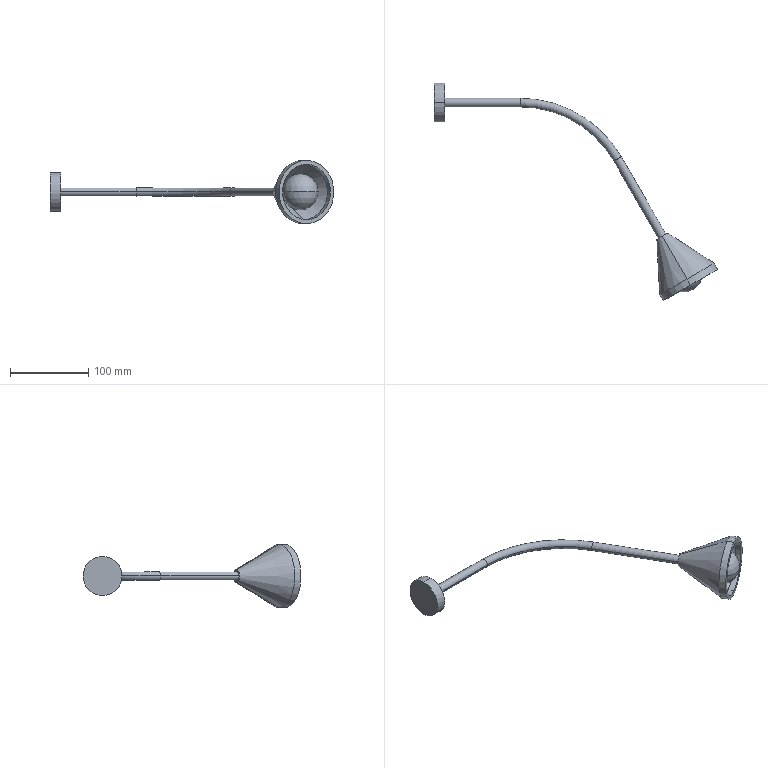Component | SolidWorks | Light-1 | 1 solid | 34 faces | box 363.07 x 279.08 x 81 mm | volume 179024 mm3 | cylinder 16 | cone 6 | plane 6 | torus 4 | sphere 2 | commonest cylinder face diameters 11 x4 1 x4 10.098 x2 71 x2 50 x2 81 x2
STEP:
#1=COLOUR_RGB('',0.7922,0.8196,0.9333);
#2=FILL_AREA_STYLE_COLOUR('',#1);
#3=FILL_AREA_STYLE('',(#2));
#4=SURFACE_STYLE_FILL_AREA(#3);
#5=SURFACE_SIDE_STYLE('',(#4));
#6=SURFACE_STYLE_USAGE(.BOTH.,#5);
#7=PRESENTATION_STYLE_ASSIGNMENT((#6));
#8=CARTESIAN_POINT('',(3.087,39.443,17.994));
#9=VERTEX_POINT('',#8);
#10=CARTESIAN_POINT('',(1.677,38.629,17.994));
#11=VERTEX_POINT('',#10);
#12=CARTESIAN_POINT('',(2.382,39.036,17.994));
#13=DIRECTION('',(0.5,-0.866,0.));
#14=DIRECTION('',(0.866,0.5,0.));
#15=AXIS2_PLACEMENT_3D('',#12,#13,#14);
#16=CIRCLE('',#15,0.8139);
#17=EDGE_CURVE('',#9,#11,#16,.T.);
#18=ORIENTED_EDGE('',*,*,#17,.T.);
#19=CARTESIAN_POINT('',(2.579,38.694,17.994));
#20=DIRECTION('',(0.,0.,-1.));
#21=DIRECTION('',(0.5611,0.8277,0.));
#22=AXIS2_PLACEMENT_3D('',#19,#20,#21);
#23=CIRCLE('',#22,0.9045);
#24=EDGE_CURVE('',#9,#11,#23,.T.);
#25=ORIENTED_EDGE('',*,*,#24,.F.);
#26=EDGE_LOOP('',(#18,#25));
#27=FACE_OUTER_BOUND('',#26,.T.);
#28=CARTESIAN_POINT('',(2.579,38.694,17.994));
#29=DIRECTION('',(0.,0.,1.));
#30=DIRECTION('',(-0.866,-0.5,0.));
#31=AXIS2_PLACEMENT_3D('',#28,#29,#30);
#32=SPHERICAL_SURFACE('',#31,0.9045);
#33=ADVANCED_FACE('',(#27),#32,.T.);
#34=ORIENTED_EDGE('',*,*,#24,.T.);
#35=CARTESIAN_POINT('',(2.382,39.036,17.994));
#36=DIRECTION('',(-0.5,0.866,0.));
#37=DIRECTION('',(0.866,0.5,0.));
#38=AXIS2_PLACEMENT_3D('',#35,#36,#37);
#39=CIRCLE('',#38,0.8139);
#40=EDGE_CURVE('',#9,#11,#39,.T.);
#41=ORIENTED_EDGE('',*,*,#40,.F.);
#42=EDGE_LOOP('',(#34,#41));
#43=FACE_OUTER_BOUND('',#42,.T.);
#44=CARTESIAN_POINT('',(2.579,38.694,17.994));
#45=DIRECTION('',(0.,0.,1.));
#46=DIRECTION('',(-0.866,-0.5,0.));
#47=AXIS2_PLACEMENT_3D('',#44,#45,#46);
#48=SPHERICAL_SURFACE('',#47,0.9045);
#49=ADVANCED_FACE('',(#43),#48,.T.);
#50=ORIENTED_EDGE('',*,*,#40,.T.);
#51=CARTESIAN_POINT('',(1.576,40.035,17.994));
#52=VERTEX_POINT('',#51);
#53=CARTESIAN_POINT('',(1.576,40.035,17.994));
#54=DIRECTION('',(0.07208,-0.9974,0.));
#55=VECTOR('',#54,39.37);
#56=LINE('',#53,#55);
#57=EDGE_CURVE('',#52,#11,#56,.T.);
#58=ORIENTED_EDGE('',*,*,#57,.F.);
#59=CARTESIAN_POINT('',(1.92,40.234,17.994));
#60=VERTEX_POINT('',#59);
#61=CARTESIAN_POINT('',(1.748,40.135,17.994));
#62=DIRECTION('',(-0.5,0.866,0.));
#63=DIRECTION('',(0.866,0.5,0.));
#64=AXIS2_PLACEMENT_3D('',#61,#62,#63);
#65=CIRCLE('',#64,0.1988);
#66=EDGE_CURVE('',#60,#52,#65,.T.);
#67=ORIENTED_EDGE('',*,*,#66,.F.);
#68=CARTESIAN_POINT('',(1.92,40.234,17.994));
#69=DIRECTION('',(0.8277,-0.5611,0.));
#70=VECTOR('',#69,39.37);
#71=LINE('',#68,#70);
#72=EDGE_CURVE('',#60,#9,#71,.T.);
#73=ORIENTED_EDGE('',*,*,#72,.T.);
#74=EDGE_LOOP('',(#50,#58,#67,#73));
#75=FACE_OUTER_BOUND('',#74,.T.);
#76=CARTESIAN_POINT('',(1.735,40.157,17.994));
#77=DIRECTION('',(0.5,-0.866,0.));
#78=DIRECTION('',(0.866,0.5,0.));
#79=AXIS2_PLACEMENT_3D('',#76,#77,#78);
#80=CONICAL_SURFACE('',#79,0.1865,0.4515);
#81=ADVANCED_FACE('',(#75),#80,.T.);
#82=CARTESIAN_POINT('',(1.748,40.135,17.994));
#83=DIRECTION('',(0.5,-0.866,0.));
#84=DIRECTION('',(0.866,0.5,0.));
#85=AXIS2_PLACEMENT_3D('',#82,#83,#84);
#86=CIRCLE('',#85,0.1988);
#87=EDGE_CURVE('',#60,#52,#86,.T.);
#88=ORIENTED_EDGE('',*,*,#87,.T.);
#89=ORIENTED_EDGE('',*,*,#57,.T.);
#90=ORIENTED_EDGE('',*,*,#17,.F.);
#91=ORIENTED_EDGE('',*,*,#72,.F.);
#92=EDGE_LOOP('',(#88,#89,#90,#91));
#93=FACE_OUTER_BOUND('',#92,.T.);
#94=CARTESIAN_POINT('',(1.735,40.157,17.994));
#95=DIRECTION('',(0.5,-0.866,0.));
#96=DIRECTION('',(0.866,0.5,0.));
#97=AXIS2_PLACEMENT_3D('',#94,#95,#96);
#98=CONICAL_SURFACE('',#97,0.1865,0.4515);
#99=ADVANCED_FACE('',(#93),#98,.T.);
#100=CARTESIAN_POINT('',(1.409,40.324,17.994));
#101=VERTEX_POINT('',#100);
#102=CARTESIAN_POINT('',(1.409,40.324,17.994));
#103=DIRECTION('',(0.5,-0.866,0.));
#104=VECTOR('',#103,39.37);
#105=LINE('',#102,#104);
#106=EDGE_CURVE('',#101,#52,#105,.T.);
#107=ORIENTED_EDGE('',*,*,#106,.T.);
#108=ORIENTED_EDGE('',*,*,#87,.F.);
#109=CARTESIAN_POINT('',(1.754,40.522,17.994));
#110=VERTEX_POINT('',#109);
#111=CARTESIAN_POINT('',(1.754,40.522,17.994));
#112=DIRECTION('',(0.5,-0.866,0.));
#113=VECTOR('',#112,39.37);
#114=LINE('',#111,#113);
#115=EDGE_CURVE('',#110,#60,#114,.T.);
#116=ORIENTED_EDGE('',*,*,#115,.F.);
#117=CARTESIAN_POINT('',(1.581,40.423,18.193));
#118=VERTEX_POINT('',#117);
#119=CARTESIAN_POINT('',(1.581,40.423,17.994));
#120=DIRECTION('',(-0.5,0.866,0.));
#121=DIRECTION('',(-0.00000001,-0.00000001,1.));
#122=AXIS2_PLACEMENT_3D('',#119,#120,#121);
#123=CIRCLE('',#122,0.1988);
#124=EDGE_CURVE('',#118,#110,#123,.T.);
#125=ORIENTED_EDGE('',*,*,#124,.F.);
#126=CARTESIAN_POINT('',(1.581,40.423,17.994));
#127=DIRECTION('',(-0.5,0.866,0.));
#128=DIRECTION('',(-0.866,-0.5,0.));
#129=AXIS2_PLACEMENT_3D('',#126,#127,#128);
#130=CIRCLE('',#129,0.1988);
#131=EDGE_CURVE('',#101,#118,#130,.T.);
#132=ORIENTED_EDGE('',*,*,#131,.F.);
#133=EDGE_LOOP('',(#107,#108,#116,#125,#132));
#134=FACE_OUTER_BOUND('',#133,.T.);
#135=CARTESIAN_POINT('',(3.225,37.576,17.994));
#136=DIRECTION('',(-0.5,0.866,0.));
#137=DIRECTION('',(-0.866,-0.5,0.));
#138=AXIS2_PLACEMENT_3D('',#135,#136,#137);
#139=CYLINDRICAL_SURFACE('',#138,0.1988);
#140=ADVANCED_FACE('',(#134),#139,.T.);
#141=ORIENTED_EDGE('',*,*,#131,.T.);
#142=CARTESIAN_POINT('',(2.747,38.404,19.392));
#143=VERTEX_POINT('',#142);
#144=CARTESIAN_POINT('',(1.581,40.423,18.193));
#145=DIRECTION('',(0.4446,-0.7701,0.4573));
#146=VECTOR('',#145,39.37);
#147=LINE('',#144,#146);
#148=EDGE_CURVE('',#118,#143,#147,.T.);
#149=ORIENTED_EDGE('',*,*,#148,.T.);
#150=CARTESIAN_POINT('',(2.747,38.404,16.597));
#151=VERTEX_POINT('',#150);
#152=CARTESIAN_POINT('',(2.747,38.404,17.994));
#153=DIRECTION('',(-0.5,0.866,0.));
#154=DIRECTION('',(0.,0.,-1.));
#155=AXIS2_PLACEMENT_3D('',#152,#153,#154);
#156=CIRCLE('',#155,1.398);
#157=EDGE_CURVE('',#151,#143,#156,.T.);
#158=ORIENTED_EDGE('',*,*,#157,.F.);
#159=CARTESIAN_POINT('',(1.581,40.423,17.796));
#160=VERTEX_POINT('',#159);
#161=CARTESIAN_POINT('',(1.581,40.423,17.796));
#162=DIRECTION('',(0.4446,-0.7701,-0.4573));
#163=VECTOR('',#162,39.37);
#164=LINE('',#161,#163);
#165=EDGE_CURVE('',#160,#151,#164,.T.);
#166=ORIENTED_EDGE('',*,*,#165,.F.);
#167=CARTESIAN_POINT('',(1.581,40.423,17.994));
#168=DIRECTION('',(-0.5,0.866,0.));
#169=DIRECTION('',(0.00000001,0.00000001,-1.));
#170=AXIS2_PLACEMENT_3D('',#167,#168,#169);
#171=CIRCLE('',#170,0.1988);
#172=EDGE_CURVE('',#160,#101,#171,.T.);
#173=ORIENTED_EDGE('',*,*,#172,.T.);
#174=EDGE_LOOP('',(#141,#149,#158,#166,#173));
#175=FACE_OUTER_BOUND('',#174,.T.);
#176=CARTESIAN_POINT('',(1.558,40.463,17.994));
#177=DIRECTION('',(0.5,-0.866,0.));
#178=DIRECTION('',(0.,0.,1.));
#179=AXIS2_PLACEMENT_3D('',#176,#177,#178);
#180=CONICAL_SURFACE('',#179,0.1748,0.475);
#181=ADVANCED_FACE('',(#175),#180,.F.);
#182=ORIENTED_EDGE('',*,*,#115,.T.);
#183=ORIENTED_EDGE('',*,*,#66,.T.);
#184=ORIENTED_EDGE('',*,*,#106,.F.);
#185=ORIENTED_EDGE('',*,*,#172,.F.);
#186=CARTESIAN_POINT('',(1.581,40.423,17.994));
#187=DIRECTION('',(-0.5,0.866,0.));
#188=DIRECTION('',(0.866,0.5,0.));
#189=AXIS2_PLACEMENT_3D('',#186,#187,#188);
#190=CIRCLE('',#189,0.1988);
#191=EDGE_CURVE('',#110,#160,#190,.T.);
#192=ORIENTED_EDGE('',*,*,#191,.F.);
#193=EDGE_LOOP('',(#182,#183,#184,#185,#192));
#194=FACE_OUTER_BOUND('',#193,.T.);
#195=CARTESIAN_POINT('',(3.225,37.576,17.994));
#196=DIRECTION('',(-0.5,0.866,0.));
#197=DIRECTION('',(-0.866,-0.5,0.));
#198=AXIS2_PLACEMENT_3D('',#195,#196,#197);
#199=CYLINDRICAL_SURFACE('',#198,0.1988);
#200=ADVANCED_FACE('',(#194),#199,.T.);
#201=ORIENTED_EDGE('',*,*,#165,.T.);
#202=CARTESIAN_POINT('',(2.747,38.404,17.994));
#203=DIRECTION('',(-0.5,0.866,0.));
#204=DIRECTION('',(0.00000001,0.,1.));
#205=AXIS2_PLACEMENT_3D('',#202,#203,#204);
#206=CIRCLE('',#205,1.398);
#207=EDGE_CURVE('',#143,#151,#206,.T.);
#208=ORIENTED_EDGE('',*,*,#207,.F.);
#209=ORIENTED_EDGE('',*,*,#148,.F.);
#210=ORIENTED_EDGE('',*,*,#124,.T.);
#211=ORIENTED_EDGE('',*,*,#191,.T.);
#212=EDGE_LOOP('',(#201,#208,#209,#210,#211));
#213=FACE_OUTER_BOUND('',#212,.T.);
#214=CARTESIAN_POINT('',(1.558,40.463,17.994));
#215=DIRECTION('',(0.5,-0.866,0.));
#216=DIRECTION('',(0.,0.,1.));
#217=AXIS2_PLACEMENT_3D('',#214,#215,#216);
#218=CONICAL_SURFACE('',#217,0.1748,0.475);
#219=ADVANCED_FACE('',(#213),#218,.F.);
#220=CARTESIAN_POINT('',(2.9,38.139,19.392));
#221=VERTEX_POINT('',#220);
#222=CARTESIAN_POINT('',(2.9,38.139,19.392));
#223=DIRECTION('',(-0.5,0.866,0.));
#224=VECTOR('',#223,39.37);
#225=LINE('',#222,#224);
#226=EDGE_CURVE('',#221,#143,#225,.T.);
#227=ORIENTED_EDGE('',*,*,#226,.T.);
#228=ORIENTED_EDGE('',*,*,#207,.T.);
#229=CARTESIAN_POINT('',(2.9,38.139,16.597));
#230=VERTEX_POINT('',#229);
#231=CARTESIAN_POINT('',(2.9,38.139,16.597));
#232=DIRECTION('',(-0.5,0.866,0.));
#233=VECTOR('',#232,39.37);
#234=LINE('',#231,#233);
#235=EDGE_CURVE('',#230,#151,#234,.T.);
#236=ORIENTED_EDGE('',*,*,#235,.F.);
#237=CARTESIAN_POINT('',(2.9,38.139,17.994));
#238=DIRECTION('',(0.5,-0.866,0.));
#239=DIRECTION('',(0.,0.,-1.));
#240=AXIS2_PLACEMENT_3D('',#237,#238,#239);
#241=CIRCLE('',#240,1.398);
#242=EDGE_CURVE('',#230,#221,#241,.T.);
#243=ORIENTED_EDGE('',*,*,#242,.T.);
#244=EDGE_LOOP('',(#227,#228,#236,#243));
#245=FACE_OUTER_BOUND('',#244,.T.);
#246=CARTESIAN_POINT('',(2.9,38.139,17.994));
#247=DIRECTION('',(0.5,-0.866,0.));
#248=DIRECTION('',(0.,0.,-1.));
#249=AXIS2_PLACEMENT_3D('',#246,#247,#248);
#250=CYLINDRICAL_SURFACE('',#249,1.398);
#251=ADVANCED_FACE('',(#245),#250,.F.);
#252=CARTESIAN_POINT('',(-5.688,47.561,17.994));
#253=VERTEX_POINT('',#252);
#254=CARTESIAN_POINT('',(-0.5905,44.618,17.994));
#255=VERTEX_POINT('',#254);
#256=CARTESIAN_POINT('',(-5.688,41.675,17.994));
#257=DIRECTION('',(0.,0.,-1.));
#258=DIRECTION('',(0.,1.,0.));
#259=AXIS2_PLACEMENT_3D('',#256,#257,#258);
#260=CIRCLE('',#259,5.886);
#261=EDGE_CURVE('',#253,#255,#260,.T.);
#262=ORIENTED_EDGE('',*,*,#261,.T.);
#263=CARTESIAN_POINT('',(-0.9656,44.401,17.994));
#264=VERTEX_POINT('',#263);
#265=CARTESIAN_POINT('',(-0.7781,44.51,17.994));
#266=DIRECTION('',(0.5,-0.866,0.));
#267=DIRECTION('',(-0.866,-0.5,0.));
#268=AXIS2_PLACEMENT_3D('',#265,#266,#267);
#269=CIRCLE('',#268,0.2165);
#270=EDGE_CURVE('',#264,#255,#269,.T.);
#271=ORIENTED_EDGE('',*,*,#270,.F.);
#272=CARTESIAN_POINT('',(-5.688,47.128,17.994));
#273=VERTEX_POINT('',#272);
#274=CARTESIAN_POINT('',(-5.688,41.675,17.994));
#275=DIRECTION('',(0.,0.,-1.));
#276=DIRECTION('',(0.,1.,0.));
#277=AXIS2_PLACEMENT_3D('',#274,#275,#276);
#278=CIRCLE('',#277,5.453);
#279=EDGE_CURVE('',#273,#264,#278,.T.);
#280=ORIENTED_EDGE('',*,*,#279,.F.);
#281=CARTESIAN_POINT('',(-5.688,47.344,17.994));
#282=DIRECTION('',(1.,0.,0.));
#283=DIRECTION('',(0.,-1.,0.));
#284=AXIS2_PLACEMENT_3D('',#281,#282,#283);
#285=CIRCLE('',#284,0.2165);
#286=EDGE_CURVE('',#273,#253,#285,.T.);
#287=ORIENTED_EDGE('',*,*,#286,.T.);
#288=EDGE_LOOP('',(#262,#271,#280,#287));
#289=FACE_OUTER_BOUND('',#288,.T.);
#290=CARTESIAN_POINT('',(-5.688,41.675,17.994));
#291=DIRECTION('',(0.,0.,-1.));
#292=DIRECTION('',(0.,-1.,0.));
#293=AXIS2_PLACEMENT_3D('',#290,#291,#292);
#294=TOROIDAL_SURFACE('',#293,5.669,0.2165);
#295=ADVANCED_FACE('',(#289),#294,.T.);
#296=CARTESIAN_POINT('',(-9.501,47.561,17.994));
#297=VERTEX_POINT('',#296);
#298=CARTESIAN_POINT('',(-9.501,47.561,17.994));
#299=DIRECTION('',(1.,0.,0.));
#300=VECTOR('',#299,39.37);
#301=LINE('',#298,#300);
#302=EDGE_CURVE('',#297,#253,#301,.T.);
#303=ORIENTED_EDGE('',*,*,#302,.T.);
#304=ORIENTED_EDGE('',*,*,#286,.F.);
#305=CARTESIAN_POINT('',(-9.501,47.128,17.994));
#306=VERTEX_POINT('',#305);
#307=CARTESIAN_POINT('',(-9.501,47.128,17.994));
#308=DIRECTION('',(1.,0.,0.));
#309=VECTOR('',#308,39.37);
#310=LINE('',#307,#309);
#311=EDGE_CURVE('',#306,#273,#310,.T.);
#312=ORIENTED_EDGE('',*,*,#311,.F.);
#313=CARTESIAN_POINT('',(-9.501,47.344,17.994));
#314=DIRECTION('',(1.,0.,0.));
#315=DIRECTION('',(0.,-1.,0.));
#316=AXIS2_PLACEMENT_3D('',#313,#314,#315);
#317=CIRCLE('',#316,0.2165);
#318=EDGE_CURVE('',#306,#297,#317,.T.);
#319=ORIENTED_EDGE('',*,*,#318,.T.);
#320=EDGE_LOOP('',(#303,#304,#312,#319));
#321=FACE_OUTER_BOUND('',#320,.T.);
#322=CARTESIAN_POINT('',(-9.501,47.344,17.994));
#323=DIRECTION('',(1.,0.,0.));
#324=DIRECTION('',(0.,-1.,0.));
#325=AXIS2_PLACEMENT_3D('',#322,#323,#324);
#326=CYLINDRICAL_SURFACE('',#325,0.2165);
#327=ADVANCED_FACE('',(#321),#326,.T.);
#328=CARTESIAN_POINT('',(-10.013,47.344,17.01));
#329=VERTEX_POINT('',#328);
#330=CARTESIAN_POINT('',(-10.013,47.344,18.979));
#331=VERTEX_POINT('',#330);
#332=CARTESIAN_POINT('',(-10.013,47.344,17.994));
#333=DIRECTION('',(-1.,0.,0.));
#334=DIRECTION('',(0.,0.,-1.));
#335=AXIS2_PLACEMENT_3D('',#332,#333,#334);
#336=CIRCLE('',#335,0.9843);
#337=EDGE_CURVE('',#329,#331,#336,.T.);
#338=ORIENTED_EDGE('',*,*,#337,.T.);
#339=CARTESIAN_POINT('',(-10.013,47.344,17.994));
#340=DIRECTION('',(-1.,0.,0.));
#341=DIRECTION('',(0.,0.,1.));
#342=AXIS2_PLACEMENT_3D('',#339,#340,#341);
#343=CIRCLE('',#342,0.9843);
#344=EDGE_CURVE('',#331,#329,#343,.T.);
#345=ORIENTED_EDGE('',*,*,#344,.T.);
#346=EDGE_LOOP('',(#338,#345));
#347=FACE_OUTER_BOUND('',#346,.T.);
#348=CARTESIAN_POINT('',(-10.013,47.344,17.994));
#349=DIRECTION('',(-1.,0.,0.));
#350=DIRECTION('',(0.,0.,1.));
#351=AXIS2_PLACEMENT_3D('',#348,#349,#350);
#352=PLANE('',#351);
#353=ADVANCED_FACE('',(#347),#352,.T.);
#354=CARTESIAN_POINT('',(-9.501,47.344,18.979));
#355=VERTEX_POINT('',#354);
#356=CARTESIAN_POINT('',(-9.501,47.344,18.979));
#357=DIRECTION('',(-1.,0.,0.));
#358=VECTOR('',#357,39.37);
#359=LINE('',#356,#358);
#360=EDGE_CURVE('',#355,#331,#359,.T.);
#361=ORIENTED_EDGE('',*,*,#360,.T.);
#362=ORIENTED_EDGE('',*,*,#337,.F.);
#363=CARTESIAN_POINT('',(-9.501,47.344,17.01));
#364=VERTEX_POINT('',#363);
#365=CARTESIAN_POINT('',(-9.501,47.344,17.01));
#366=DIRECTION('',(-1.,0.,0.));
#367=VECTOR('',#366,39.37);
#368=LINE('',#365,#367);
#369=EDGE_CURVE('',#364,#329,#368,.T.);
#370=ORIENTED_EDGE('',*,*,#369,.F.);
#371=CARTESIAN_POINT('',(-9.501,47.344,17.994));
#372=DIRECTION('',(-1.,0.,0.));
#373=DIRECTION('',(0.,0.,-1.));
#374=AXIS2_PLACEMENT_3D('',#371,#372,#373);
#375=CIRCLE('',#374,0.9843);
#376=EDGE_CURVE('',#364,#355,#375,.T.);
#377=ORIENTED_EDGE('',*,*,#376,.T.);
#378=EDGE_LOOP('',(#361,#362,#370,#377));
#379=FACE_OUTER_BOUND('',#378,.T.);
#380=CARTESIAN_POINT('',(-9.501,47.344,17.994));
#381=DIRECTION('',(-1.,0.,0.));
#382=DIRECTION('',(0.,0.,1.));
#383=AXIS2_PLACEMENT_3D('',#380,#381,#382);
#384=CYLINDRICAL_SURFACE('',#383,0.9843);
#385=ADVANCED_FACE('',(#379),#384,.T.);
#386=ORIENTED_EDGE('',*,*,#369,.T.);
#387=ORIENTED_EDGE('',*,*,#344,.F.);
#388=ORIENTED_EDGE('',*,*,#360,.F.);
#389=CARTESIAN_POINT('',(-9.501,47.344,17.994));
#390=DIRECTION('',(-1.,0.,0.));
#391=DIRECTION('',(0.,0.,1.));
#392=AXIS2_PLACEMENT_3D('',#389,#390,#391);
#393=CIRCLE('',#392,0.9843);
#394=EDGE_CURVE('',#355,#364,#393,.T.);
#395=ORIENTED_EDGE('',*,*,#394,.T.);
#396=EDGE_LOOP('',(#386,#387,#388,#395));
#397=FACE_OUTER_BOUND('',#396,.T.);
#398=CARTESIAN_POINT('',(-9.501,47.344,17.994));
#399=DIRECTION('',(-1.,0.,0.));
#400=DIRECTION('',(0.,0.,1.));
#401=AXIS2_PLACEMENT_3D('',#398,#399,#400);
#402=CYLINDRICAL_SURFACE('',#401,0.9843);
#403=ADVANCED_FACE('',(#397),#402,.T.);
#404=CARTESIAN_POINT('',(-9.501,47.344,17.994));
#405=DIRECTION('',(1.,0.,0.));
#406=DIRECTION('',(0.,1.,0.));
#407=AXIS2_PLACEMENT_3D('',#404,#405,#406);
#408=CIRCLE('',#407,0.2165);
#409=EDGE_CURVE('',#297,#306,#408,.T.);
#410=ORIENTED_EDGE('',*,*,#409,.F.);
#411=ORIENTED_EDGE('',*,*,#318,.F.);
#412=EDGE_LOOP('',(#410,#411));
#413=FACE_BOUND('',#412,.T.);
#414=ORIENTED_EDGE('',*,*,#376,.F.);
#415=ORIENTED_EDGE('',*,*,#394,.F.);
#416=EDGE_LOOP('',(#414,#415));
#417=FACE_OUTER_BOUND('',#416,.T.);
#418=CARTESIAN_POINT('',(-9.501,47.344,17.994));
#419=DIRECTION('',(-1.,0.,0.));
#420=DIRECTION('',(0.,0.,1.));
#421=AXIS2_PLACEMENT_3D('',#418,#419,#420);
#422=PLANE('',#421);
#423=ADVANCED_FACE('',(#413,#417),#422,.F.);
#424=ORIENTED_EDGE('',*,*,#311,.T.);
#425=CARTESIAN_POINT('',(-5.688,47.344,17.994));
#426=DIRECTION('',(1.,0.,0.));
#427=DIRECTION('',(0.,1.,0.));
#428=AXIS2_PLACEMENT_3D('',#425,#426,#427);
#429=CIRCLE('',#428,0.2165);
#430=EDGE_CURVE('',#253,#273,#429,.T.);
#431=ORIENTED_EDGE('',*,*,#430,.F.);
#432=ORIENTED_EDGE('',*,*,#302,.F.);
#433=ORIENTED_EDGE('',*,*,#409,.T.);
#434=EDGE_LOOP('',(#424,#431,#432,#433));
#435=FACE_OUTER_BOUND('',#434,.T.);
#436=CARTESIAN_POINT('',(-9.501,47.344,17.994));
#437=DIRECTION('',(1.,0.,0.));
#438=DIRECTION('',(0.,-1.,0.));
#439=AXIS2_PLACEMENT_3D('',#436,#437,#438);
#440=CYLINDRICAL_SURFACE('',#439,0.2165);
#441=ADVANCED_FACE('',(#435),#440,.T.);
#442=ORIENTED_EDGE('',*,*,#279,.T.);
#443=CARTESIAN_POINT('',(-0.7781,44.51,17.994));
#444=DIRECTION('',(0.5,-0.866,0.));
#445=DIRECTION('',(0.866,0.5,0.));
#446=AXIS2_PLACEMENT_3D('',#443,#444,#445);
#447=CIRCLE('',#446,0.2165);
#448=EDGE_CURVE('',#255,#264,#447,.T.);
#449=ORIENTED_EDGE('',*,*,#448,.F.);
#450=ORIENTED_EDGE('',*,*,#261,.F.);
#451=ORIENTED_EDGE('',*,*,#430,.T.);
#452=EDGE_LOOP('',(#442,#449,#450,#451));
#453=FACE_OUTER_BOUND('',#452,.T.);
#454=CARTESIAN_POINT('',(-5.688,41.675,17.994));
#455=DIRECTION('',(0.,0.,-1.));
#456=DIRECTION('',(0.,-1.,0.));
#457=AXIS2_PLACEMENT_3D('',#454,#455,#456);
#458=TOROIDAL_SURFACE('',#457,5.669,0.2165);
#459=ADVANCED_FACE('',(#453),#458,.T.);
#460=CARTESIAN_POINT('',(1.671,40.702,17.994));
#461=VERTEX_POINT('',#460);
#462=CARTESIAN_POINT('',(-0.5905,44.618,17.994));
#463=DIRECTION('',(0.5,-0.866,0.));
#464=VECTOR('',#463,39.37);
#465=LINE('',#462,#464);
#466=EDGE_CURVE('',#255,#461,#465,.T.);
#467=ORIENTED_EDGE('',*,*,#466,.F.);
#468=ORIENTED_EDGE('',*,*,#448,.T.);
#469=CARTESIAN_POINT('',(1.295,40.485,17.994));
#470=VERTEX_POINT('',#469);
#471=CARTESIAN_POINT('',(-0.9656,44.401,17.994));
#472=DIRECTION('',(0.5,-0.866,0.));
#473=VECTOR('',#472,39.37);
#474=LINE('',#471,#473);
#475=EDGE_CURVE('',#264,#470,#474,.T.);
#476=ORIENTED_EDGE('',*,*,#475,.T.);
#477=CARTESIAN_POINT('',(1.483,40.593,17.994));
#478=DIRECTION('',(0.5,-0.866,0.));
#479=DIRECTION('',(0.866,0.5,0.));
#480=AXIS2_PLACEMENT_3D('',#477,#478,#479);
#481=CIRCLE('',#480,0.2165);
#482=EDGE_CURVE('',#461,#470,#481,.T.);
#483=ORIENTED_EDGE('',*,*,#482,.F.);
#484=EDGE_LOOP('',(#467,#468,#476,#483));
#485=FACE_OUTER_BOUND('',#484,.T.);
#486=CARTESIAN_POINT('',(-0.7781,44.51,17.994));
#487=DIRECTION('',(0.5,-0.866,0.));
#488=DIRECTION('',(-0.866,-0.5,0.));
#489=AXIS2_PLACEMENT_3D('',#486,#487,#488);
#490=CYLINDRICAL_SURFACE('',#489,0.2165);
#491=ADVANCED_FACE('',(#485),#490,.T.);
#492=ORIENTED_EDGE('',*,*,#475,.F.);
#493=ORIENTED_EDGE('',*,*,#270,.T.);
#494=ORIENTED_EDGE('',*,*,#466,.T.);
#495=CARTESIAN_POINT('',(1.483,40.593,17.994));
#496=DIRECTION('',(0.5,-0.866,0.));
#497=DIRECTION('',(-0.866,-0.5,0.));
#498=AXIS2_PLACEMENT_3D('',#495,#496,#497);
#499=CIRCLE('',#498,0.2165);
#500=EDGE_CURVE('',#470,#461,#499,.T.);
#501=ORIENTED_EDGE('',*,*,#500,.F.);
#502=EDGE_LOOP('',(#492,#493,#494,#501));
#503=FACE_OUTER_BOUND('',#502,.T.);
#504=CARTESIAN_POINT('',(-0.7781,44.51,17.994));
#505=DIRECTION('',(0.5,-0.866,0.));
#506=DIRECTION('',(-0.866,-0.5,0.));
#507=AXIS2_PLACEMENT_3D('',#504,#505,#506);
#508=CYLINDRICAL_SURFACE('',#507,0.2165);
#509=ADVANCED_FACE('',(#503),#508,.T.);
#510=CARTESIAN_POINT('',(2.9,38.139,16.4));
#511=VERTEX_POINT('',#510);
#512=CARTESIAN_POINT('',(2.723,38.445,16.4));
#513=VERTEX_POINT('',#512);
#514=CARTESIAN_POINT('',(2.9,38.139,16.4));
#515=DIRECTION('',(-0.5,0.866,0.));
#516=VECTOR('',#515,39.37);
#517=LINE('',#514,#516);
#518=EDGE_CURVE('',#511,#513,#517,.T.);
#519=ORIENTED_EDGE('',*,*,#518,.F.);
#520=CARTESIAN_POINT('',(2.9,38.139,19.589));
#521=VERTEX_POINT('',#520);
#522=CARTESIAN_POINT('',(2.9,38.139,17.994));
#523=DIRECTION('',(0.5,-0.866,0.));
#524=DIRECTION('',(0.,0.,1.));
#525=AXIS2_PLACEMENT_3D('',#522,#523,#524);
#526=CIRCLE('',#525,1.594);
#527=EDGE_CURVE('',#521,#511,#526,.T.);
#528=ORIENTED_EDGE('',*,*,#527,.F.);
#529=CARTESIAN_POINT('',(2.723,38.445,19.589));
#530=VERTEX_POINT('',#529);
#531=CARTESIAN_POINT('',(2.9,38.139,19.589));
#532=DIRECTION('',(-0.5,0.866,0.));
#533=VECTOR('',#532,39.37);
#534=LINE('',#531,#533);
#535=EDGE_CURVE('',#521,#530,#534,.T.);
#536=ORIENTED_EDGE('',*,*,#535,.T.);
#537=CARTESIAN_POINT('',(2.723,38.445,17.994));
#538=DIRECTION('',(-0.5,0.866,0.));
#539=DIRECTION('',(0.,0.,-1.));
#540=AXIS2_PLACEMENT_3D('',#537,#538,#539);
#541=CIRCLE('',#540,1.594);
#542=EDGE_CURVE('',#513,#530,#541,.T.);
#543=ORIENTED_EDGE('',*,*,#542,.F.);
#544=EDGE_LOOP('',(#519,#528,#536,#543));
#545=FACE_OUTER_BOUND('',#544,.T.);
#546=CARTESIAN_POINT('',(2.9,38.139,17.994));
#547=DIRECTION('',(0.5,-0.866,0.));
#548=DIRECTION('',(0.,0.,-1.));
#549=AXIS2_PLACEMENT_3D('',#546,#547,#548);
#550=CYLINDRICAL_SURFACE('',#549,1.594);
#551=ADVANCED_FACE('',(#545),#550,.T.);
#552=CARTESIAN_POINT('',(1.483,40.593,17.676));
#553=VERTEX_POINT('',#552);
#554=CARTESIAN_POINT('',(1.483,40.593,17.676));
#555=DIRECTION('',(0.4446,-0.7701,-0.4573));
#556=VECTOR('',#555,39.37);
#557=LINE('',#554,#556);
#558=EDGE_CURVE('',#553,#513,#557,.T.);
#559=ORIENTED_EDGE('',*,*,#558,.T.);
#560=ORIENTED_EDGE('',*,*,#542,.T.);
#561=CARTESIAN_POINT('',(1.483,40.593,18.313));
#562=VERTEX_POINT('',#561);
#563=CARTESIAN_POINT('',(1.483,40.593,18.313));
#564=DIRECTION('',(0.4446,-0.7701,0.4573));
#565=VECTOR('',#564,39.37);
#566=LINE('',#563,#565);
#567=EDGE_CURVE('',#562,#530,#566,.T.);
#568=ORIENTED_EDGE('',*,*,#567,.F.);
#569=CARTESIAN_POINT('',(1.483,40.593,17.994));
#570=DIRECTION('',(-0.5,0.866,0.));
#571=DIRECTION('',(0.,0.,-1.));
#572=AXIS2_PLACEMENT_3D('',#569,#570,#571);
#573=CIRCLE('',#572,0.3189);
#574=EDGE_CURVE('',#553,#562,#573,.T.);
#575=ORIENTED_EDGE('',*,*,#574,.F.);
#576=EDGE_LOOP('',(#559,#560,#568,#575));
#577=FACE_OUTER_BOUND('',#576,.T.);
#578=CARTESIAN_POINT('',(1.458,40.636,17.994));
#579=DIRECTION('',(0.5,-0.866,0.));
#580=DIRECTION('',(0.,0.,1.));
#581=AXIS2_PLACEMENT_3D('',#578,#579,#580);
#582=CONICAL_SURFACE('',#581,0.2934,0.475);
#583=ADVANCED_FACE('',(#577),#582,.T.);
#584=ORIENTED_EDGE('',*,*,#482,.T.);
#585=ORIENTED_EDGE('',*,*,#500,.T.);
#586=EDGE_LOOP('',(#584,#585));
#587=FACE_BOUND('',#586,.T.);
#588=CARTESIAN_POINT('',(1.483,40.593,17.994));
#589=DIRECTION('',(-0.5,0.866,0.));
#590=DIRECTION('',(0.,0.,1.));
#591=AXIS2_PLACEMENT_3D('',#588,#589,#590);
#592=CIRCLE('',#591,0.3189);
#593=EDGE_CURVE('',#562,#553,#592,.T.);
#594=ORIENTED_EDGE('',*,*,#593,.T.);
#595=ORIENTED_EDGE('',*,*,#574,.T.);
#596=EDGE_LOOP('',(#594,#595));
#597=FACE_OUTER_BOUND('',#596,.T.);
#598=CARTESIAN_POINT('',(-3.832,37.525,17.994));
#599=DIRECTION('',(0.5,-0.866,0.));
#600=DIRECTION('',(0.,0.,-1.));
#601=AXIS2_PLACEMENT_3D('',#598,#599,#600);
#602=PLANE('',#601);
#603=ADVANCED_FACE('',(#587,#597),#602,.F.);
#604=ORIENTED_EDGE('',*,*,#567,.T.);
#605=CARTESIAN_POINT('',(2.723,38.445,17.994));
#606=DIRECTION('',(-0.5,0.866,0.));
#607=DIRECTION('',(0.,0.,1.));
#608=AXIS2_PLACEMENT_3D('',#605,#606,#607);
#609=CIRCLE('',#608,1.594);
#610=EDGE_CURVE('',#530,#513,#609,.T.);
#611=ORIENTED_EDGE('',*,*,#610,.T.);
#612=ORIENTED_EDGE('',*,*,#558,.F.);
#613=ORIENTED_EDGE('',*,*,#593,.F.);
#614=EDGE_LOOP('',(#604,#611,#612,#613));
#615=FACE_OUTER_BOUND('',#614,.T.);
#616=CARTESIAN_POINT('',(1.458,40.636,17.994));
#617=DIRECTION('',(0.5,-0.866,0.));
#618=DIRECTION('',(0.,0.,1.));
#619=AXIS2_PLACEMENT_3D('',#616,#617,#618);
#620=CONICAL_SURFACE('',#619,0.2934,0.475);
#621=ADVANCED_FACE('',(#615),#620,.T.);
#622=ORIENTED_EDGE('',*,*,#535,.F.);
#623=CARTESIAN_POINT('',(2.9,38.139,17.994));
#624=DIRECTION('',(0.5,-0.866,0.));
#625=DIRECTION('',(0.,0.,-1.));
#626=AXIS2_PLACEMENT_3D('',#623,#624,#625);
#627=CIRCLE('',#626,1.594);
#628=EDGE_CURVE('',#511,#521,#627,.T.);
#629=ORIENTED_EDGE('',*,*,#628,.F.);
#630=ORIENTED_EDGE('',*,*,#518,.T.);
#631=ORIENTED_EDGE('',*,*,#610,.F.);
#632=EDGE_LOOP('',(#622,#629,#630,#631));
#633=FACE_OUTER_BOUND('',#632,.T.);
#634=CARTESIAN_POINT('',(2.9,38.139,17.994));
#635=DIRECTION('',(0.5,-0.866,0.));
#636=DIRECTION('',(0.,0.,-1.));
#637=AXIS2_PLACEMENT_3D('',#634,#635,#636);
#638=CYLINDRICAL_SURFACE('',#637,1.594);
#639=ADVANCED_FACE('',(#633),#638,.T.);
#640=CARTESIAN_POINT('',(2.9,38.139,17.994));
#641=DIRECTION('',(0.5,-0.866,0.));
#642=DIRECTION('',(0.,0.,1.));
#643=AXIS2_PLACEMENT_3D('',#640,#641,#642);
#644=CIRCLE('',#643,1.398);
#645=EDGE_CURVE('',#221,#230,#644,.T.);
#646=ORIENTED_EDGE('',*,*,#645,.F.);
#647=ORIENTED_EDGE('',*,*,#242,.F.);
#648=EDGE_LOOP('',(#646,#647));
#649=FACE_BOUND('',#648,.T.);
#650=ORIENTED_EDGE('',*,*,#527,.T.);
#651=ORIENTED_EDGE('',*,*,#628,.T.);
#652=EDGE_LOOP('',(#650,#651));
#653=FACE_OUTER_BOUND('',#652,.T.);
#654=CARTESIAN_POINT('',(2.9,38.139,17.994));
#655=DIRECTION('',(0.5,-0.866,0.));
#656=DIRECTION('',(-0.866,-0.5,0.));
#657=AXIS2_PLACEMENT_3D('',#654,#655,#656);
#658=PLANE('',#657);
#659=ADVANCED_FACE('',(#649,#653),#658,.T.);
#660=ORIENTED_EDGE('',*,*,#235,.T.);
#661=ORIENTED_EDGE('',*,*,#157,.T.);
#662=ORIENTED_EDGE('',*,*,#226,.F.);
#663=ORIENTED_EDGE('',*,*,#645,.T.);
#664=EDGE_LOOP('',(#660,#661,#662,#663));
#665=FACE_OUTER_BOUND('',#664,.T.);
#666=CARTESIAN_POINT('',(2.9,38.139,17.994));
#667=DIRECTION('',(0.5,-0.866,0.));
#668=DIRECTION('',(0.,0.,-1.));
#669=AXIS2_PLACEMENT_3D('',#666,#667,#668);
#670=CYLINDRICAL_SURFACE('',#669,1.398);
#671=ADVANCED_FACE('',(#665),#670,.F.);
#672=CLOSED_SHELL('',(#33,#49,#81,#99,#140,#181,#200,#219,#251,#295,#327,#353,#385,#403,#423,#441,#459,#491,#509,#551,#583,#603,#621,#639,#659,#671));
#673=CARTESIAN_POINT('',(-5.688,47.325,17.994));
#674=VERTEX_POINT('',#673);
#675=CARTESIAN_POINT('',(-0.7951,44.5,17.994));
#676=VERTEX_POINT('',#675);
#677=CARTESIAN_POINT('',(-5.688,41.675,17.994));
#678=DIRECTION('',(0.,0.,-1.));
#679=DIRECTION('',(0.,1.,0.));
#680=AXIS2_PLACEMENT_3D('',#677,#678,#679);
#681=CIRCLE('',#680,5.65);
#682=EDGE_CURVE('',#674,#676,#681,.T.);
#683=ORIENTED_EDGE('',*,*,#682,.T.);
#684=CARTESIAN_POINT('',(-0.761,44.52,17.994));
#685=VERTEX_POINT('',#684);
#686=CARTESIAN_POINT('',(-0.7781,44.51,17.994));
#687=DIRECTION('',(0.5,-0.866,0.));
#688=DIRECTION('',(-0.866,-0.5,0.));
#689=AXIS2_PLACEMENT_3D('',#686,#687,#688);
#690=CIRCLE('',#689,0.01969);
#691=EDGE_CURVE('',#676,#685,#690,.T.);
#692=ORIENTED_EDGE('',*,*,#691,.T.);
#693=CARTESIAN_POINT('',(-5.688,47.364,17.994));
#694=VERTEX_POINT('',#693);
#695=CARTESIAN_POINT('',(-5.688,41.675,17.994));
#696=DIRECTION('',(0.,0.,-1.));
#697=DIRECTION('',(0.,1.,0.));
#698=AXIS2_PLACEMENT_3D('',#695,#696,#697);
#699=CIRCLE('',#698,5.689);
#700=EDGE_CURVE('',#694,#685,#699,.T.);
#701=ORIENTED_EDGE('',*,*,#700,.F.);
#702=CARTESIAN_POINT('',(-5.688,47.344,17.994));
#703=DIRECTION('',(1.,0.,0.));
#704=DIRECTION('',(0.,-1.,0.));
#705=AXIS2_PLACEMENT_3D('',#702,#703,#704);
#706=CIRCLE('',#705,0.01969);
#707=EDGE_CURVE('',#674,#694,#706,.T.);
#708=ORIENTED_EDGE('',*,*,#707,.F.);
#709=EDGE_LOOP('',(#683,#692,#701,#708));
#710=FACE_OUTER_BOUND('',#709,.T.);
#711=CARTESIAN_POINT('',(-5.688,41.675,17.994));
#712=DIRECTION('',(0.,0.,-1.));
#713=DIRECTION('',(0.,-1.,0.));
#714=AXIS2_PLACEMENT_3D('',#711,#712,#713);
#715=TOROIDAL_SURFACE('',#714,5.669,0.01969);
#716=ADVANCED_FACE('',(#710),#715,.F.);
#717=CARTESIAN_POINT('',(-9.304,47.325,17.994));
#718=VERTEX_POINT('',#717);
#719=CARTESIAN_POINT('',(-9.304,47.325,17.994));
#720=DIRECTION('',(1.,0.,0.));
#721=VECTOR('',#720,39.37);
#722=LINE('',#719,#721);
#723=EDGE_CURVE('',#718,#674,#722,.T.);
#724=ORIENTED_EDGE('',*,*,#723,.T.);
#725=ORIENTED_EDGE('',*,*,#707,.T.);
#726=CARTESIAN_POINT('',(-9.304,47.364,17.994));
#727=VERTEX_POINT('',#726);
#728=CARTESIAN_POINT('',(-9.304,47.364,17.994));
#729=DIRECTION('',(1.,0.,0.));
#730=VECTOR('',#729,39.37);
#731=LINE('',#728,#730);
#732=EDGE_CURVE('',#727,#694,#731,.T.);
#733=ORIENTED_EDGE('',*,*,#732,.F.);
#734=CARTESIAN_POINT('',(-9.304,47.344,17.994));
#735=DIRECTION('',(1.,0.,0.));
#736=DIRECTION('',(0.,-1.,0.));
#737=AXIS2_PLACEMENT_3D('',#734,#735,#736);
#738=CIRCLE('',#737,0.01969);
#739=EDGE_CURVE('',#718,#727,#738,.T.);
#740=ORIENTED_EDGE('',*,*,#739,.F.);
#741=EDGE_LOOP('',(#724,#725,#733,#740));
#742=FACE_OUTER_BOUND('',#741,.T.);
#743=CARTESIAN_POINT('',(-9.501,47.344,17.994));
#744=DIRECTION('',(1.,0.,0.));
#745=DIRECTION('',(0.,-1.,0.));
#746=AXIS2_PLACEMENT_3D('',#743,#744,#745);
#747=CYLINDRICAL_SURFACE('',#746,0.01969);
#748=ADVANCED_FACE('',(#742),#747,.F.);
#749=CARTESIAN_POINT('',(-9.304,47.344,17.994));
#750=DIRECTION('',(1.,0.,0.));
#751=DIRECTION('',(0.,1.,0.));
#752=AXIS2_PLACEMENT_3D('',#749,#750,#751);
#753=CIRCLE('',#752,0.01969);
#754=EDGE_CURVE('',#727,#718,#753,.T.);
#755=ORIENTED_EDGE('',*,*,#754,.T.);
#756=ORIENTED_EDGE('',*,*,#739,.T.);
#757=EDGE_LOOP('',(#755,#756));
#758=FACE_OUTER_BOUND('',#757,.T.);
#759=CARTESIAN_POINT('',(-9.304,47.344,17.994));
#760=DIRECTION('',(1.,0.,0.));
#761=DIRECTION('',(0.,-1.,0.));
#762=AXIS2_PLACEMENT_3D('',#759,#760,#761);
#763=PLANE('',#762);
#764=ADVANCED_FACE('',(#758),#763,.T.);
#765=ORIENTED_EDGE('',*,*,#732,.T.);
#766=CARTESIAN_POINT('',(-5.688,47.344,17.994));
#767=DIRECTION('',(1.,0.,0.));
#768=DIRECTION('',(0.,1.,0.));
#769=AXIS2_PLACEMENT_3D('',#766,#767,#768);
#770=CIRCLE('',#769,0.01969);
#771=EDGE_CURVE('',#694,#674,#770,.T.);
#772=ORIENTED_EDGE('',*,*,#771,.T.);
#773=ORIENTED_EDGE('',*,*,#723,.F.);
#774=ORIENTED_EDGE('',*,*,#754,.F.);
#775=EDGE_LOOP('',(#765,#772,#773,#774));
#776=FACE_OUTER_BOUND('',#775,.T.);
#777=CARTESIAN_POINT('',(-9.501,47.344,17.994));
#778=DIRECTION('',(1.,0.,0.));
#779=DIRECTION('',(0.,-1.,0.));
#780=AXIS2_PLACEMENT_3D('',#777,#778,#779);
#781=CYLINDRICAL_SURFACE('',#780,0.01969);
#782=ADVANCED_FACE('',(#776),#781,.F.);
#783=ORIENTED_EDGE('',*,*,#700,.T.);
#784=CARTESIAN_POINT('',(-0.7781,44.51,17.994));
#785=DIRECTION('',(0.5,-0.866,0.));
#786=DIRECTION('',(0.866,0.5,0.));
#787=AXIS2_PLACEMENT_3D('',#784,#785,#786);
#788=CIRCLE('',#787,0.01969);
#789=EDGE_CURVE('',#685,#676,#788,.T.);
#790=ORIENTED_EDGE('',*,*,#789,.T.);
#791=ORIENTED_EDGE('',*,*,#682,.F.);
#792=ORIENTED_EDGE('',*,*,#771,.F.);
#793=EDGE_LOOP('',(#783,#790,#791,#792));
#794=FACE_OUTER_BOUND('',#793,.T.);
#795=CARTESIAN_POINT('',(-5.688,41.675,17.994));
#796=DIRECTION('',(0.,0.,-1.));
#797=DIRECTION('',(0.,-1.,0.));
#798=AXIS2_PLACEMENT_3D('',#795,#796,#797);
#799=TOROIDAL_SURFACE('',#798,5.669,0.01969);
#800=ADVANCED_FACE('',(#794),#799,.F.);
#801=CARTESIAN_POINT('',(1.564,40.413,17.994));
#802=VERTEX_POINT('',#801);
#803=CARTESIAN_POINT('',(-0.7951,44.5,17.994));
#804=DIRECTION('',(0.5,-0.866,0.));
#805=VECTOR('',#804,39.37);
#806=LINE('',#803,#805);
#807=EDGE_CURVE('',#676,#802,#806,.T.);
#808=ORIENTED_EDGE('',*,*,#807,.F.);
#809=ORIENTED_EDGE('',*,*,#789,.F.);
#810=CARTESIAN_POINT('',(1.598,40.433,17.994));
#811=VERTEX_POINT('',#810);
#812=CARTESIAN_POINT('',(-0.761,44.52,17.994));
#813=DIRECTION('',(0.5,-0.866,0.));
#814=VECTOR('',#813,39.37);
#815=LINE('',#812,#814);
#816=EDGE_CURVE('',#685,#811,#815,.T.);
#817=ORIENTED_EDGE('',*,*,#816,.T.);
#818=CARTESIAN_POINT('',(1.581,40.423,17.994));
#819=DIRECTION('',(0.5,-0.866,0.));
#820=DIRECTION('',(0.866,0.5,0.));
#821=AXIS2_PLACEMENT_3D('',#818,#819,#820);
#822=CIRCLE('',#821,0.01969);
#823=EDGE_CURVE('',#811,#802,#822,.T.);
#824=ORIENTED_EDGE('',*,*,#823,.T.);
#825=EDGE_LOOP('',(#808,#809,#817,#824));
#826=FACE_OUTER_BOUND('',#825,.T.);
#827=CARTESIAN_POINT('',(-0.7781,44.51,17.994));
#828=DIRECTION('',(0.5,-0.866,0.));
#829=DIRECTION('',(-0.866,-0.5,0.));
#830=AXIS2_PLACEMENT_3D('',#827,#828,#829);
#831=CYLINDRICAL_SURFACE('',#830,0.01969);
#832=ADVANCED_FACE('',(#826),#831,.F.);
#833=ORIENTED_EDGE('',*,*,#816,.F.);
#834=ORIENTED_EDGE('',*,*,#691,.F.);
#835=ORIENTED_EDGE('',*,*,#807,.T.);
#836=CARTESIAN_POINT('',(1.581,40.423,17.994));
#837=DIRECTION('',(0.5,-0.866,0.));
#838=DIRECTION('',(-0.866,-0.5,0.));
#839=AXIS2_PLACEMENT_3D('',#836,#837,#838);
#840=CIRCLE('',#839,0.01969);
#841=EDGE_CURVE('',#802,#811,#840,.T.);
#842=ORIENTED_EDGE('',*,*,#841,.T.);
#843=EDGE_LOOP('',(#833,#834,#835,#842));
#844=FACE_OUTER_BOUND('',#843,.T.);
#845=CARTESIAN_POINT('',(-0.7781,44.51,17.994));
#846=DIRECTION('',(0.5,-0.866,0.));
#847=DIRECTION('',(-0.866,-0.5,0.));
#848=AXIS2_PLACEMENT_3D('',#845,#846,#847);
#849=CYLINDRICAL_SURFACE('',#848,0.01969);
#850=ADVANCED_FACE('',(#844),#849,.F.);
#851=ORIENTED_EDGE('',*,*,#823,.F.);
#852=ORIENTED_EDGE('',*,*,#841,.F.);
#853=EDGE_LOOP('',(#851,#852));
#854=FACE_OUTER_BOUND('',#853,.T.);
#855=CARTESIAN_POINT('',(1.581,40.423,17.994));
#856=DIRECTION('',(-0.5,0.866,0.));
#857=DIRECTION('',(-0.866,-0.5,0.));
#858=AXIS2_PLACEMENT_3D('',#855,#856,#857);
#859=PLANE('',#858);
#860=ADVANCED_FACE('',(#854),#859,.T.);
#861=CLOSED_SHELL('',(#716,#748,#764,#782,#800,#832,#850,#860));
#862=ORIENTED_CLOSED_SHELL('',*,#861,.F.);
#863=BREP_WITH_VOIDS('',#672,(#862));
#864=STYLED_ITEM('',(#7),#863);
#865=PRESENTATION_LAYER_ASSIGNMENT('','',(#864));
#866=CARTESIAN_POINT('',(0.,0.,0.));
#867=DIRECTION('',(0.,0.,1.));
#868=DIRECTION('',(1.,0.,0.));
#869=AXIS2_PLACEMENT_3D('',#866,#867,#868);
#870=(LENGTH_UNIT()NAMED_UNIT(*)SI_UNIT($,.METRE.));
#871=LENGTH_MEASURE_WITH_UNIT(LENGTH_MEASURE(0.0254),#870);
#872=DIMENSIONAL_EXPONENTS(1.,0.,0.,0.,0.,0.,0.);
#873=(CONVERSION_BASED_UNIT('',#871)LENGTH_UNIT()NAMED_UNIT(#872));
#874=UNCERTAINTY_MEASURE_WITH_UNIT(LENGTH_MEASURE(0.00001),#873,'','');
#875=(NAMED_UNIT(*)PLANE_ANGLE_UNIT()SI_UNIT($,.RADIAN.));
#876=(NAMED_UNIT(*)SI_UNIT($,.STERADIAN.)SOLID_ANGLE_UNIT());
#877=(GEOMETRIC_REPRESENTATION_CONTEXT(3)GLOBAL_UNCERTAINTY_ASSIGNED_CONTEXT((#874))GLOBAL_UNIT_ASSIGNED_CONTEXT((#873,#875,#876))REPRESENTATION_CONTEXT('',''));
#878=ADVANCED_BREP_SHAPE_REPRESENTATION('',(#863,#869),#877);
#879=(LENGTH_UNIT()NAMED_UNIT(*)SI_UNIT($,.METRE.));
#880=LENGTH_MEASURE_WITH_UNIT(LENGTH_MEASURE(0.0254),#879);
#881=DIMENSIONAL_EXPONENTS(1.,0.,0.,0.,0.,0.,0.);
#882=(CONVERSION_BASED_UNIT('',#880)LENGTH_UNIT()NAMED_UNIT(#881));
#883=UNCERTAINTY_MEASURE_WITH_UNIT(LENGTH_MEASURE(0.00001),#882,'','');
#884=(NAMED_UNIT(*)PLANE_ANGLE_UNIT()SI_UNIT($,.RADIAN.));
#885=(NAMED_UNIT(*)SI_UNIT($,.STERADIAN.)SOLID_ANGLE_UNIT());
#886=(GEOMETRIC_REPRESENTATION_CONTEXT(3)GLOBAL_UNCERTAINTY_ASSIGNED_CONTEXT((#883))GLOBAL_UNIT_ASSIGNED_CONTEXT((#882,#884,#885))REPRESENTATION_CONTEXT('',''));
#887=MECHANICAL_DESIGN_GEOMETRIC_PRESENTATION_REPRESENTATION('',(#864),#886);